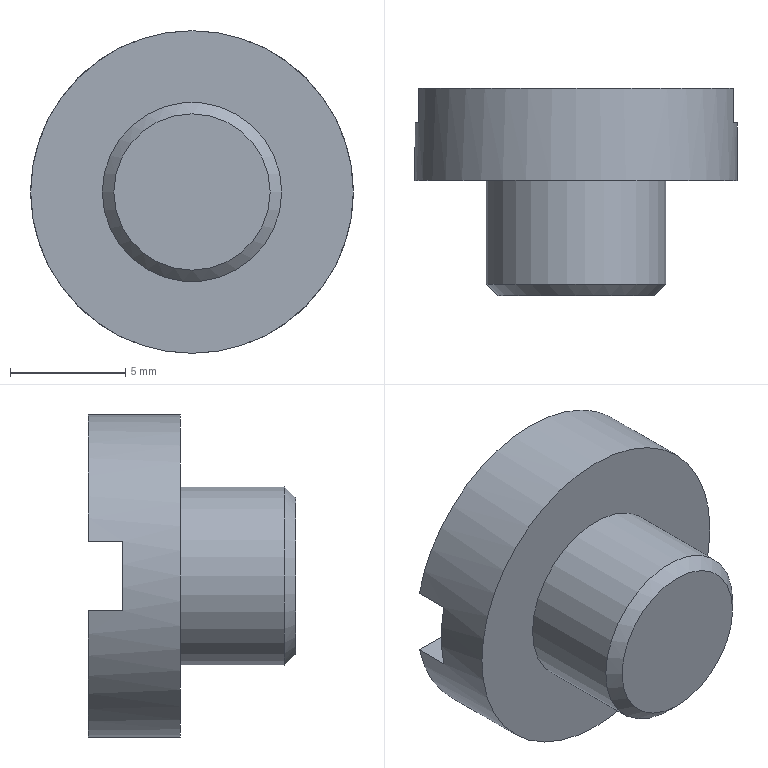Component | NX | BOLT_M8X5 | 1 solid | 10 faces | volume 788 mm3 | plane 7 | cylinder 2 | cone 1 | commonest cylinder face diameters 7.785 x1 14 x1